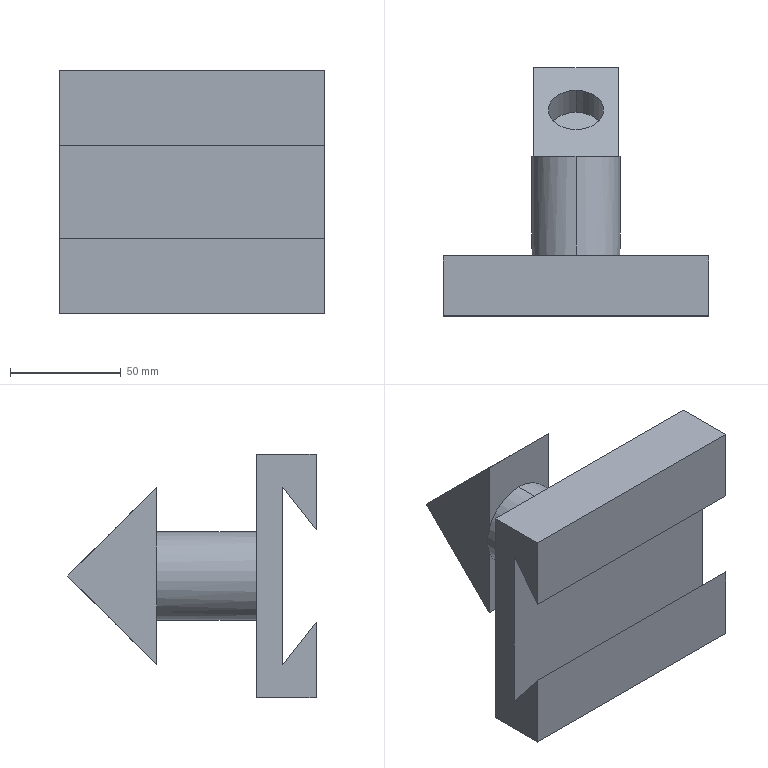Component | SolidWorks | PassiveRollerAssembly-1_DovetailSlot-1 | 1 solid | 26 faces | box 120 x 112 x 110 mm | volume 350204 mm3 | plane 20 | cylinder 6 | commonest cylinder face diameters 25 x4 40 x2
build123d program:
from build123d import *

# Parameters (mm, degrees)
BOSS_EXTRUDE1_DEPTH = 120
SKETCH2_R           = 20
BOSS_EXTRUDE2_DEPTH = 45
BOSS_EXTRUDE3_DEPTH = 19
SKETCH4_R           = 12.5
CUT_EXTRUDE1_DEPTH  = 14


with BuildPart() as part:
    # Sketch1 → Boss-Extrude1 (new body)
    with BuildSketch(Plane.XY):
        Polygon((-55, 0), (55, 0), (55, -27), (21, -27), (40, -12), (-40, -12), (-21, -27), (-55, -27), align=None)
    extrude(amount=BOSS_EXTRUDE1_DEPTH)

    # Sketch2 → Boss-Extrude2 (add)
    with BuildSketch(Plane(origin=(0, 0, 0), x_dir=(1, 0, 0), z_dir=(0, 1, 0))):
        with Locations((0, -60)):
            Circle(SKETCH2_R)
    extrude(amount=BOSS_EXTRUDE2_DEPTH)

    # Sketch3 → Boss-Extrude3 (add, symmetric)
    with BuildSketch(Plane.XY.offset(60)):
        Polygon((-40, 45), (40, 45), (0, 85), align=None)
    extrude(amount=BOSS_EXTRUDE3_DEPTH, both=True)

    # Sketch4 → Cut-Extrude1 (cut)
    with BuildSketch(Plane(origin=(42.5, 42.5, 0), x_dir=(0, 0, -1), z_dir=(0.7071, 0.7071, 0))):
        with Locations(Location((-60, 33.154, 0), (0, 0, 90))):
            Circle(SKETCH4_R)
    cut_extrude1 = extrude(amount=-CUT_EXTRUDE1_DEPTH, mode=Mode.SUBTRACT)

    # Mirror1: Cut-Extrude1 across plane
    add(cut_extrude1.mirror(Plane(origin=(0, 0, 0), x_dir=(0, 0, 1), z_dir=(1, 0, 0))), mode=Mode.SUBTRACT)


solid = part.part

# Placed as in the assembly
solid = solid.moved(Location((2156.026, 589, 269.5), (0, 90, 0)))
STEP:
#1=CARTESIAN_POINT('',(87.245,25.047,11.319));
#2=VERTEX_POINT('',#1);
#3=CARTESIAN_POINT('',(87.245,25.743,10.623));
#4=VERTEX_POINT('',#3);
#5=CARTESIAN_POINT('',(87.245,25.395,10.971));
#6=DIRECTION('',(0.,-0.7071,-0.7071));
#7=DIRECTION('',(0.,0.7071,-0.7071));
#8=AXIS2_PLACEMENT_3D('',#5,#6,#7);
#9=CIRCLE('',#8,0.4921);
#10=EDGE_CURVE('',#2,#4,#9,.T.);
#11=ORIENTED_EDGE('',*,*,#10,.T.);
#12=CARTESIAN_POINT('',(87.245,26.133,11.013));
#13=VERTEX_POINT('',#12);
#14=CARTESIAN_POINT('',(87.245,25.743,10.623));
#15=DIRECTION('',(0.,0.7071,0.7071));
#16=VECTOR('',#15,39.37);
#17=LINE('',#14,#16);
#18=EDGE_CURVE('',#4,#13,#17,.T.);
#19=ORIENTED_EDGE('',*,*,#18,.T.);
#20=CARTESIAN_POINT('',(87.245,25.437,11.708));
#21=VERTEX_POINT('',#20);
#22=CARTESIAN_POINT('',(87.245,25.785,11.36));
#23=DIRECTION('',(0.,-0.7071,-0.7071));
#24=DIRECTION('',(0.,0.7071,-0.7071));
#25=AXIS2_PLACEMENT_3D('',#22,#23,#24);
#26=CIRCLE('',#25,0.4921);
#27=EDGE_CURVE('',#21,#13,#26,.T.);
#28=ORIENTED_EDGE('',*,*,#27,.F.);
#29=CARTESIAN_POINT('',(87.245,25.047,11.319));
#30=DIRECTION('',(0.,0.7071,0.7071));
#31=VECTOR('',#30,39.37);
#32=LINE('',#29,#31);
#33=EDGE_CURVE('',#2,#21,#32,.T.);
#34=ORIENTED_EDGE('',*,*,#33,.F.);
#35=EDGE_LOOP('',(#11,#19,#28,#34));
#36=FACE_OUTER_BOUND('',#35,.T.);
#37=CARTESIAN_POINT('',(87.245,25.395,10.971));
#38=DIRECTION('',(0.,0.7071,0.7071));
#39=DIRECTION('',(0.,-0.7071,0.7071));
#40=AXIS2_PLACEMENT_3D('',#37,#38,#39);
#41=CYLINDRICAL_SURFACE('',#40,0.4921);
#42=ADVANCED_FACE('',(#36),#41,.F.);
#43=CARTESIAN_POINT('',(87.245,25.047,9.902));
#44=VERTEX_POINT('',#43);
#45=CARTESIAN_POINT('',(87.245,25.743,10.598));
#46=VERTEX_POINT('',#45);
#47=CARTESIAN_POINT('',(87.245,25.395,10.25));
#48=DIRECTION('',(0.,0.7071,-0.7071));
#49=DIRECTION('',(0.,0.7071,0.7071));
#50=AXIS2_PLACEMENT_3D('',#47,#48,#49);
#51=CIRCLE('',#50,0.4921);
#52=EDGE_CURVE('',#44,#46,#51,.T.);
#53=ORIENTED_EDGE('',*,*,#52,.F.);
#54=CARTESIAN_POINT('',(87.245,25.437,9.512));
#55=VERTEX_POINT('',#54);
#56=CARTESIAN_POINT('',(87.245,25.047,9.902));
#57=DIRECTION('',(0.,0.7071,-0.7071));
#58=VECTOR('',#57,39.37);
#59=LINE('',#56,#58);
#60=EDGE_CURVE('',#44,#55,#59,.T.);
#61=ORIENTED_EDGE('',*,*,#60,.T.);
#62=CARTESIAN_POINT('',(87.245,26.133,10.208));
#63=VERTEX_POINT('',#62);
#64=CARTESIAN_POINT('',(87.245,25.785,9.86));
#65=DIRECTION('',(0.,0.7071,-0.7071));
#66=DIRECTION('',(0.,0.7071,0.7071));
#67=AXIS2_PLACEMENT_3D('',#64,#65,#66);
#68=CIRCLE('',#67,0.4921);
#69=EDGE_CURVE('',#55,#63,#68,.T.);
#70=ORIENTED_EDGE('',*,*,#69,.T.);
#71=CARTESIAN_POINT('',(87.245,25.743,10.598));
#72=DIRECTION('',(0.,0.7071,-0.7071));
#73=VECTOR('',#72,39.37);
#74=LINE('',#71,#73);
#75=EDGE_CURVE('',#46,#63,#74,.T.);
#76=ORIENTED_EDGE('',*,*,#75,.F.);
#77=EDGE_LOOP('',(#53,#61,#70,#76));
#78=FACE_OUTER_BOUND('',#77,.T.);
#79=CARTESIAN_POINT('',(87.245,25.395,10.25));
#80=DIRECTION('',(0.,0.7071,-0.7071));
#81=DIRECTION('',(0.,0.7071,0.7071));
#82=AXIS2_PLACEMENT_3D('',#79,#80,#81);
#83=CYLINDRICAL_SURFACE('',#82,0.4921);
#84=ADVANCED_FACE('',(#78),#83,.F.);
#85=CARTESIAN_POINT('',(87.245,24.961,11.398));
#86=VERTEX_POINT('',#85);
#87=CARTESIAN_POINT('',(87.993,24.961,10.856));
#88=VERTEX_POINT('',#87);
#89=CARTESIAN_POINT('',(87.245,24.961,10.61));
#90=DIRECTION('',(0.,1.,-0.));
#91=DIRECTION('',(0.,0.,1.));
#92=AXIS2_PLACEMENT_3D('',#89,#90,#91);
#93=CIRCLE('',#92,0.7874);
#94=EDGE_CURVE('',#86,#88,#93,.T.);
#95=ORIENTED_EDGE('',*,*,#94,.F.);
#96=CARTESIAN_POINT('',(87.245,23.189,11.398));
#97=VERTEX_POINT('',#96);
#98=CARTESIAN_POINT('',(87.245,24.961,11.398));
#99=DIRECTION('',(0.,-1.,0.));
#100=VECTOR('',#99,39.37);
#101=LINE('',#98,#100);
#102=EDGE_CURVE('',#86,#97,#101,.T.);
#103=ORIENTED_EDGE('',*,*,#102,.T.);
#104=CARTESIAN_POINT('',(87.245,23.189,9.823));
#105=VERTEX_POINT('',#104);
#106=CARTESIAN_POINT('',(87.245,23.189,10.61));
#107=DIRECTION('',(0.,1.,-0.));
#108=DIRECTION('',(0.,0.,-1.));
#109=AXIS2_PLACEMENT_3D('',#106,#107,#108);
#110=CIRCLE('',#109,0.7874);
#111=EDGE_CURVE('',#97,#105,#110,.T.);
#112=ORIENTED_EDGE('',*,*,#111,.T.);
#113=CARTESIAN_POINT('',(87.245,24.961,9.823));
#114=VERTEX_POINT('',#113);
#115=CARTESIAN_POINT('',(87.245,24.961,9.823));
#116=DIRECTION('',(0.,-1.,0.));
#117=VECTOR('',#116,39.37);
#118=LINE('',#115,#117);
#119=EDGE_CURVE('',#114,#105,#118,.T.);
#120=ORIENTED_EDGE('',*,*,#119,.F.);
#121=CARTESIAN_POINT('',(87.993,24.961,10.364));
#122=VERTEX_POINT('',#121);
#123=CARTESIAN_POINT('',(87.245,24.961,10.61));
#124=DIRECTION('',(0.,1.,-0.));
#125=DIRECTION('',(0.,0.,1.));
#126=AXIS2_PLACEMENT_3D('',#123,#124,#125);
#127=CIRCLE('',#126,0.7874);
#128=EDGE_CURVE('',#122,#114,#127,.T.);
#129=ORIENTED_EDGE('',*,*,#128,.F.);
#130=CARTESIAN_POINT('',(87.245,24.961,10.61));
#131=DIRECTION('',(0.,1.,-0.));
#132=DIRECTION('',(0.,0.,1.));
#133=AXIS2_PLACEMENT_3D('',#130,#131,#132);
#134=CIRCLE('',#133,0.7874);
#135=EDGE_CURVE('',#88,#122,#134,.T.);
#136=ORIENTED_EDGE('',*,*,#135,.F.);
#137=EDGE_LOOP('',(#95,#103,#112,#120,#129,#136));
#138=FACE_OUTER_BOUND('',#137,.T.);
#139=CARTESIAN_POINT('',(87.245,24.961,10.61));
#140=DIRECTION('',(0.,-1.,0.));
#141=DIRECTION('',(0.,0.,-1.));
#142=AXIS2_PLACEMENT_3D('',#139,#140,#141);
#143=CYLINDRICAL_SURFACE('',#142,0.7874);
#144=ADVANCED_FACE('',(#138),#143,.T.);
#145=CARTESIAN_POINT('',(86.497,26.535,10.61));
#146=VERTEX_POINT('',#145);
#147=CARTESIAN_POINT('',(86.497,24.961,12.185));
#148=VERTEX_POINT('',#147);
#149=CARTESIAN_POINT('',(86.497,24.961,12.185));
#150=DIRECTION('',(0.,-0.7071,0.7071));
#151=VECTOR('',#150,39.37);
#152=LINE('',#149,#151);
#153=EDGE_CURVE('',#146,#148,#152,.T.);
#154=ORIENTED_EDGE('',*,*,#153,.T.);
#155=CARTESIAN_POINT('',(87.993,24.961,12.185));
#156=VERTEX_POINT('',#155);
#157=CARTESIAN_POINT('',(87.993,24.961,12.185));
#158=DIRECTION('',(-1.,0.,0.));
#159=VECTOR('',#158,39.37);
#160=LINE('',#157,#159);
#161=EDGE_CURVE('',#156,#148,#160,.T.);
#162=ORIENTED_EDGE('',*,*,#161,.F.);
#163=CARTESIAN_POINT('',(87.993,26.535,10.61));
#164=VERTEX_POINT('',#163);
#165=CARTESIAN_POINT('',(87.993,24.961,12.185));
#166=DIRECTION('',(0.,-0.7071,0.7071));
#167=VECTOR('',#166,39.37);
#168=LINE('',#165,#167);
#169=EDGE_CURVE('',#164,#156,#168,.T.);
#170=ORIENTED_EDGE('',*,*,#169,.F.);
#171=CARTESIAN_POINT('',(87.993,26.535,10.61));
#172=DIRECTION('',(-1.,0.,0.));
#173=VECTOR('',#172,39.37);
#174=LINE('',#171,#173);
#175=EDGE_CURVE('',#164,#146,#174,.T.);
#176=ORIENTED_EDGE('',*,*,#175,.T.);
#177=EDGE_LOOP('',(#154,#162,#170,#176));
#178=FACE_OUTER_BOUND('',#177,.T.);
#179=ORIENTED_EDGE('',*,*,#27,.T.);
#180=CARTESIAN_POINT('',(87.245,25.785,11.36));
#181=DIRECTION('',(0.,-0.7071,-0.7071));
#182=DIRECTION('',(0.,0.7071,-0.7071));
#183=AXIS2_PLACEMENT_3D('',#180,#181,#182);
#184=CIRCLE('',#183,0.4921);
#185=EDGE_CURVE('',#13,#21,#184,.T.);
#186=ORIENTED_EDGE('',*,*,#185,.T.);
#187=EDGE_LOOP('',(#179,#186));
#188=FACE_BOUND('',#187,.T.);
#189=CARTESIAN_POINT('',(87.993,24.961,12.185));
#190=DIRECTION('',(0.,-0.7071,-0.7071));
#191=DIRECTION('',(0.,0.7071,-0.7071));
#192=AXIS2_PLACEMENT_3D('',#189,#190,#191);
#193=PLANE('',#192);
#194=ADVANCED_FACE('',(#178,#188),#193,.F.);
#195=CARTESIAN_POINT('',(86.497,24.961,10.364));
#196=VERTEX_POINT('',#195);
#197=CARTESIAN_POINT('',(86.497,24.961,10.856));
#198=VERTEX_POINT('',#197);
#199=CARTESIAN_POINT('',(87.245,24.961,10.61));
#200=DIRECTION('',(0.,1.,-0.));
#201=DIRECTION('',(0.,0.,1.));
#202=AXIS2_PLACEMENT_3D('',#199,#200,#201);
#203=CIRCLE('',#202,0.7874);
#204=EDGE_CURVE('',#196,#198,#203,.T.);
#205=ORIENTED_EDGE('',*,*,#204,.T.);
#206=CARTESIAN_POINT('',(86.497,24.961,12.185));
#207=DIRECTION('',(0.,-0.,-1.));
#208=VECTOR('',#207,39.37);
#209=LINE('',#206,#208);
#210=EDGE_CURVE('',#198,#196,#209,.T.);
#211=ORIENTED_EDGE('',*,*,#210,.T.);
#212=EDGE_LOOP('',(#205,#211));
#213=FACE_OUTER_BOUND('',#212,.T.);
#214=CARTESIAN_POINT('',(87.245,24.961,10.61));
#215=DIRECTION('',(0.,1.,0.));
#216=DIRECTION('',(0.,-0.,1.));
#217=AXIS2_PLACEMENT_3D('',#214,#215,#216);
#218=PLANE('',#217);
#219=ADVANCED_FACE('',(#213),#218,.T.);
#220=CARTESIAN_POINT('',(84.883,23.189,8.445));
#221=VERTEX_POINT('',#220);
#222=CARTESIAN_POINT('',(84.883,23.189,12.776));
#223=VERTEX_POINT('',#222);
#224=CARTESIAN_POINT('',(84.883,23.189,12.776));
#225=DIRECTION('',(0.,-0.,1.));
#226=VECTOR('',#225,39.37);
#227=LINE('',#224,#226);
#228=EDGE_CURVE('',#221,#223,#227,.T.);
#229=ORIENTED_EDGE('',*,*,#228,.T.);
#230=CARTESIAN_POINT('',(89.607,23.189,12.776));
#231=VERTEX_POINT('',#230);
#232=CARTESIAN_POINT('',(89.607,23.189,12.776));
#233=DIRECTION('',(-1.,0.,0.));
#234=VECTOR('',#233,39.37);
#235=LINE('',#232,#234);
#236=EDGE_CURVE('',#231,#223,#235,.T.);
#237=ORIENTED_EDGE('',*,*,#236,.F.);
#238=CARTESIAN_POINT('',(89.607,23.189,8.445));
#239=VERTEX_POINT('',#238);
#240=CARTESIAN_POINT('',(89.607,23.189,12.776));
#241=DIRECTION('',(0.,-0.,1.));
#242=VECTOR('',#241,39.37);
#243=LINE('',#240,#242);
#244=EDGE_CURVE('',#239,#231,#243,.T.);
#245=ORIENTED_EDGE('',*,*,#244,.F.);
#246=CARTESIAN_POINT('',(89.607,23.189,8.445));
#247=DIRECTION('',(-1.,0.,0.));
#248=VECTOR('',#247,39.37);
#249=LINE('',#246,#248);
#250=EDGE_CURVE('',#239,#221,#249,.T.);
#251=ORIENTED_EDGE('',*,*,#250,.T.);
#252=EDGE_LOOP('',(#229,#237,#245,#251));
#253=FACE_OUTER_BOUND('',#252,.T.);
#254=CARTESIAN_POINT('',(87.245,23.189,10.61));
#255=DIRECTION('',(0.,1.,-0.));
#256=DIRECTION('',(0.,0.,-1.));
#257=AXIS2_PLACEMENT_3D('',#254,#255,#256);
#258=CIRCLE('',#257,0.7874);
#259=EDGE_CURVE('',#105,#97,#258,.T.);
#260=ORIENTED_EDGE('',*,*,#259,.F.);
#261=ORIENTED_EDGE('',*,*,#111,.F.);
#262=EDGE_LOOP('',(#260,#261));
#263=FACE_BOUND('',#262,.T.);
#264=CARTESIAN_POINT('',(89.607,23.189,12.776));
#265=DIRECTION('',(0.,-1.,-0.));
#266=DIRECTION('',(0.,0.,-1.));
#267=AXIS2_PLACEMENT_3D('',#264,#265,#266);
#268=PLANE('',#267);
#269=ADVANCED_FACE('',(#253,#263),#268,.F.);
#270=CARTESIAN_POINT('',(84.883,22.126,8.445));
#271=VERTEX_POINT('',#270);
#272=CARTESIAN_POINT('',(84.883,23.189,8.445));
#273=DIRECTION('',(0.,1.,-0.));
#274=VECTOR('',#273,39.37);
#275=LINE('',#272,#274);
#276=EDGE_CURVE('',#271,#221,#275,.T.);
#277=ORIENTED_EDGE('',*,*,#276,.T.);
#278=ORIENTED_EDGE('',*,*,#250,.F.);
#279=CARTESIAN_POINT('',(89.607,22.126,8.445));
#280=VERTEX_POINT('',#279);
#281=CARTESIAN_POINT('',(89.607,23.189,8.445));
#282=DIRECTION('',(0.,1.,-0.));
#283=VECTOR('',#282,39.37);
#284=LINE('',#281,#283);
#285=EDGE_CURVE('',#280,#239,#284,.T.);
#286=ORIENTED_EDGE('',*,*,#285,.F.);
#287=CARTESIAN_POINT('',(89.607,22.126,8.445));
#288=DIRECTION('',(-1.,0.,0.));
#289=VECTOR('',#288,39.37);
#290=LINE('',#287,#289);
#291=EDGE_CURVE('',#280,#271,#290,.T.);
#292=ORIENTED_EDGE('',*,*,#291,.T.);
#293=EDGE_LOOP('',(#277,#278,#286,#292));
#294=FACE_OUTER_BOUND('',#293,.T.);
#295=CARTESIAN_POINT('',(89.607,23.189,8.445));
#296=DIRECTION('',(0.,0.,1.));
#297=DIRECTION('',(1.,0.,0.));
#298=AXIS2_PLACEMENT_3D('',#295,#296,#297);
#299=PLANE('',#298);
#300=ADVANCED_FACE('',(#294),#299,.F.);
#301=CARTESIAN_POINT('',(84.883,22.126,12.776));
#302=VERTEX_POINT('',#301);
#303=CARTESIAN_POINT('',(84.883,23.189,12.776));
#304=DIRECTION('',(0.,-1.,0.));
#305=VECTOR('',#304,39.37);
#306=LINE('',#303,#305);
#307=EDGE_CURVE('',#223,#302,#306,.T.);
#308=ORIENTED_EDGE('',*,*,#307,.T.);
#309=CARTESIAN_POINT('',(89.607,22.126,12.776));
#310=VERTEX_POINT('',#309);
#311=CARTESIAN_POINT('',(89.607,22.126,12.776));
#312=DIRECTION('',(-1.,0.,0.));
#313=VECTOR('',#312,39.37);
#314=LINE('',#311,#313);
#315=EDGE_CURVE('',#310,#302,#314,.T.);
#316=ORIENTED_EDGE('',*,*,#315,.F.);
#317=CARTESIAN_POINT('',(89.607,23.189,12.776));
#318=DIRECTION('',(0.,-1.,0.));
#319=VECTOR('',#318,39.37);
#320=LINE('',#317,#319);
#321=EDGE_CURVE('',#231,#310,#320,.T.);
#322=ORIENTED_EDGE('',*,*,#321,.F.);
#323=ORIENTED_EDGE('',*,*,#236,.T.);
#324=EDGE_LOOP('',(#308,#316,#322,#323));
#325=FACE_OUTER_BOUND('',#324,.T.);
#326=CARTESIAN_POINT('',(89.607,23.189,12.776));
#327=DIRECTION('',(0.,-0.,-1.));
#328=DIRECTION('',(-1.,0.,0.));
#329=AXIS2_PLACEMENT_3D('',#326,#327,#328);
#330=PLANE('',#329);
#331=ADVANCED_FACE('',(#325),#330,.F.);
#332=CARTESIAN_POINT('',(84.883,22.126,11.437));
#333=VERTEX_POINT('',#332);
#334=CARTESIAN_POINT('',(84.883,22.126,12.776));
#335=DIRECTION('',(0.,-0.,-1.));
#336=VECTOR('',#335,39.37);
#337=LINE('',#334,#336);
#338=EDGE_CURVE('',#302,#333,#337,.T.);
#339=ORIENTED_EDGE('',*,*,#338,.T.);
#340=CARTESIAN_POINT('',(89.607,22.126,11.437));
#341=VERTEX_POINT('',#340);
#342=CARTESIAN_POINT('',(89.607,22.126,11.437));
#343=DIRECTION('',(-1.,0.,0.));
#344=VECTOR('',#343,39.37);
#345=LINE('',#342,#344);
#346=EDGE_CURVE('',#341,#333,#345,.T.);
#347=ORIENTED_EDGE('',*,*,#346,.F.);
#348=CARTESIAN_POINT('',(89.607,22.126,12.776));
#349=DIRECTION('',(0.,-0.,-1.));
#350=VECTOR('',#349,39.37);
#351=LINE('',#348,#350);
#352=EDGE_CURVE('',#310,#341,#351,.T.);
#353=ORIENTED_EDGE('',*,*,#352,.F.);
#354=ORIENTED_EDGE('',*,*,#315,.T.);
#355=EDGE_LOOP('',(#339,#347,#353,#354));
#356=FACE_OUTER_BOUND('',#355,.T.);
#357=CARTESIAN_POINT('',(89.607,22.126,12.776));
#358=DIRECTION('',(0.,1.,-0.));
#359=DIRECTION('',(0.,0.,1.));
#360=AXIS2_PLACEMENT_3D('',#357,#358,#359);
#361=PLANE('',#360);
#362=ADVANCED_FACE('',(#356),#361,.F.);
#363=CARTESIAN_POINT('',(84.883,22.717,12.185));
#364=VERTEX_POINT('',#363);
#365=CARTESIAN_POINT('',(84.883,22.126,11.437));
#366=DIRECTION('',(0.,0.6196,0.7849));
#367=VECTOR('',#366,39.37);
#368=LINE('',#365,#367);
#369=EDGE_CURVE('',#333,#364,#368,.T.);
#370=ORIENTED_EDGE('',*,*,#369,.T.);
#371=CARTESIAN_POINT('',(89.607,22.717,12.185));
#372=VERTEX_POINT('',#371);
#373=CARTESIAN_POINT('',(89.607,22.717,12.185));
#374=DIRECTION('',(-1.,0.,0.));
#375=VECTOR('',#374,39.37);
#376=LINE('',#373,#375);
#377=EDGE_CURVE('',#372,#364,#376,.T.);
#378=ORIENTED_EDGE('',*,*,#377,.F.);
#379=CARTESIAN_POINT('',(89.607,22.126,11.437));
#380=DIRECTION('',(0.,0.6196,0.7849));
#381=VECTOR('',#380,39.37);
#382=LINE('',#379,#381);
#383=EDGE_CURVE('',#341,#372,#382,.T.);
#384=ORIENTED_EDGE('',*,*,#383,.F.);
#385=ORIENTED_EDGE('',*,*,#346,.T.);
#386=EDGE_LOOP('',(#370,#378,#384,#385));
#387=FACE_OUTER_BOUND('',#386,.T.);
#388=CARTESIAN_POINT('',(89.607,22.126,11.437));
#389=DIRECTION('',(0.,-0.7849,0.6196));
#390=DIRECTION('',(0.,-0.6196,-0.7849));
#391=AXIS2_PLACEMENT_3D('',#388,#389,#390);
#392=PLANE('',#391);
#393=ADVANCED_FACE('',(#387),#392,.F.);
#394=CARTESIAN_POINT('',(84.883,22.717,9.035));
#395=VERTEX_POINT('',#394);
#396=CARTESIAN_POINT('',(84.883,22.717,9.035));
#397=DIRECTION('',(0.,0.,-1.));
#398=VECTOR('',#397,39.37);
#399=LINE('',#396,#398);
#400=EDGE_CURVE('',#364,#395,#399,.T.);
#401=ORIENTED_EDGE('',*,*,#400,.T.);
#402=CARTESIAN_POINT('',(89.607,22.717,9.035));
#403=VERTEX_POINT('',#402);
#404=CARTESIAN_POINT('',(89.607,22.717,9.035));
#405=DIRECTION('',(-1.,0.,0.));
#406=VECTOR('',#405,39.37);
#407=LINE('',#404,#406);
#408=EDGE_CURVE('',#403,#395,#407,.T.);
#409=ORIENTED_EDGE('',*,*,#408,.F.);
#410=CARTESIAN_POINT('',(89.607,22.717,9.035));
#411=DIRECTION('',(0.,0.,-1.));
#412=VECTOR('',#411,39.37);
#413=LINE('',#410,#412);
#414=EDGE_CURVE('',#372,#403,#413,.T.);
#415=ORIENTED_EDGE('',*,*,#414,.F.);
#416=ORIENTED_EDGE('',*,*,#377,.T.);
#417=EDGE_LOOP('',(#401,#409,#415,#416));
#418=FACE_OUTER_BOUND('',#417,.T.);
#419=CARTESIAN_POINT('',(89.607,22.717,9.035));
#420=DIRECTION('',(0.,1.,0.));
#421=DIRECTION('',(0.,-0.,1.));
#422=AXIS2_PLACEMENT_3D('',#419,#420,#421);
#423=PLANE('',#422);
#424=ADVANCED_FACE('',(#418),#423,.F.);
#425=CARTESIAN_POINT('',(84.883,22.126,9.783));
#426=VERTEX_POINT('',#425);
#427=CARTESIAN_POINT('',(84.883,22.126,9.783));
#428=DIRECTION('',(0.,-0.6196,0.7849));
#429=VECTOR('',#428,39.37);
#430=LINE('',#427,#429);
#431=EDGE_CURVE('',#395,#426,#430,.T.);
#432=ORIENTED_EDGE('',*,*,#431,.T.);
#433=CARTESIAN_POINT('',(89.607,22.126,9.783));
#434=VERTEX_POINT('',#433);
#435=CARTESIAN_POINT('',(89.607,22.126,9.783));
#436=DIRECTION('',(-1.,0.,0.));
#437=VECTOR('',#436,39.37);
#438=LINE('',#435,#437);
#439=EDGE_CURVE('',#434,#426,#438,.T.);
#440=ORIENTED_EDGE('',*,*,#439,.F.);
#441=CARTESIAN_POINT('',(89.607,22.126,9.783));
#442=DIRECTION('',(0.,-0.6196,0.7849));
#443=VECTOR('',#442,39.37);
#444=LINE('',#441,#443);
#445=EDGE_CURVE('',#403,#434,#444,.T.);
#446=ORIENTED_EDGE('',*,*,#445,.F.);
#447=ORIENTED_EDGE('',*,*,#408,.T.);
#448=EDGE_LOOP('',(#432,#440,#446,#447));
#449=FACE_OUTER_BOUND('',#448,.T.);
#450=CARTESIAN_POINT('',(89.607,22.126,9.783));
#451=DIRECTION('',(0.,-0.7849,-0.6196));
#452=DIRECTION('',(0.,0.6196,-0.7849));
#453=AXIS2_PLACEMENT_3D('',#450,#451,#452);
#454=PLANE('',#453);
#455=ADVANCED_FACE('',(#449),#454,.F.);
#456=CARTESIAN_POINT('',(84.883,22.126,8.445));
#457=DIRECTION('',(0.,0.,-1.));
#458=VECTOR('',#457,39.37);
#459=LINE('',#456,#458);
#460=EDGE_CURVE('',#426,#271,#459,.T.);
#461=ORIENTED_EDGE('',*,*,#460,.T.);
#462=ORIENTED_EDGE('',*,*,#291,.F.);
#463=CARTESIAN_POINT('',(89.607,22.126,8.445));
#464=DIRECTION('',(0.,0.,-1.));
#465=VECTOR('',#464,39.37);
#466=LINE('',#463,#465);
#467=EDGE_CURVE('',#434,#280,#466,.T.);
#468=ORIENTED_EDGE('',*,*,#467,.F.);
#469=ORIENTED_EDGE('',*,*,#439,.T.);
#470=EDGE_LOOP('',(#461,#462,#468,#469));
#471=FACE_OUTER_BOUND('',#470,.T.);
#472=CARTESIAN_POINT('',(89.607,22.126,8.445));
#473=DIRECTION('',(0.,1.,0.));
#474=DIRECTION('',(0.,-0.,1.));
#475=AXIS2_PLACEMENT_3D('',#472,#473,#474);
#476=PLANE('',#475);
#477=ADVANCED_FACE('',(#471),#476,.F.);
#478=ORIENTED_EDGE('',*,*,#285,.T.);
#479=ORIENTED_EDGE('',*,*,#244,.T.);
#480=ORIENTED_EDGE('',*,*,#321,.T.);
#481=ORIENTED_EDGE('',*,*,#352,.T.);
#482=ORIENTED_EDGE('',*,*,#383,.T.);
#483=ORIENTED_EDGE('',*,*,#414,.T.);
#484=ORIENTED_EDGE('',*,*,#445,.T.);
#485=ORIENTED_EDGE('',*,*,#467,.T.);
#486=EDGE_LOOP('',(#478,#479,#480,#481,#482,#483,#484,#485));
#487=FACE_OUTER_BOUND('',#486,.T.);
#488=CARTESIAN_POINT('',(89.607,23.189,10.61));
#489=DIRECTION('',(-1.,0.,0.));
#490=DIRECTION('',(0.,0.,1.));
#491=AXIS2_PLACEMENT_3D('',#488,#489,#490);
#492=PLANE('',#491);
#493=ADVANCED_FACE('',(#487),#492,.F.);
#494=ORIENTED_EDGE('',*,*,#276,.F.);
#495=ORIENTED_EDGE('',*,*,#460,.F.);
#496=ORIENTED_EDGE('',*,*,#431,.F.);
#497=ORIENTED_EDGE('',*,*,#400,.F.);
#498=ORIENTED_EDGE('',*,*,#369,.F.);
#499=ORIENTED_EDGE('',*,*,#338,.F.);
#500=ORIENTED_EDGE('',*,*,#307,.F.);
#501=ORIENTED_EDGE('',*,*,#228,.F.);
#502=EDGE_LOOP('',(#494,#495,#496,#497,#498,#499,#500,#501));
#503=FACE_OUTER_BOUND('',#502,.T.);
#504=CARTESIAN_POINT('',(84.883,23.189,10.61));
#505=DIRECTION('',(-1.,0.,0.));
#506=DIRECTION('',(0.,0.,1.));
#507=AXIS2_PLACEMENT_3D('',#504,#505,#506);
#508=PLANE('',#507);
#509=ADVANCED_FACE('',(#503),#508,.T.);
#510=ORIENTED_EDGE('',*,*,#102,.F.);
#511=CARTESIAN_POINT('',(87.245,24.961,10.61));
#512=DIRECTION('',(0.,1.,-0.));
#513=DIRECTION('',(0.,0.,1.));
#514=AXIS2_PLACEMENT_3D('',#511,#512,#513);
#515=CIRCLE('',#514,0.7874);
#516=EDGE_CURVE('',#198,#86,#515,.T.);
#517=ORIENTED_EDGE('',*,*,#516,.F.);
#518=ORIENTED_EDGE('',*,*,#204,.F.);
#519=CARTESIAN_POINT('',(87.245,24.961,10.61));
#520=DIRECTION('',(0.,1.,-0.));
#521=DIRECTION('',(0.,0.,1.));
#522=AXIS2_PLACEMENT_3D('',#519,#520,#521);
#523=CIRCLE('',#522,0.7874);
#524=EDGE_CURVE('',#114,#196,#523,.T.);
#525=ORIENTED_EDGE('',*,*,#524,.F.);
#526=ORIENTED_EDGE('',*,*,#119,.T.);
#527=ORIENTED_EDGE('',*,*,#259,.T.);
#528=EDGE_LOOP('',(#510,#517,#518,#525,#526,#527));
#529=FACE_OUTER_BOUND('',#528,.T.);
#530=CARTESIAN_POINT('',(87.245,24.961,10.61));
#531=DIRECTION('',(0.,-1.,0.));
#532=DIRECTION('',(0.,0.,-1.));
#533=AXIS2_PLACEMENT_3D('',#530,#531,#532);
#534=CYLINDRICAL_SURFACE('',#533,0.7874);
#535=ADVANCED_FACE('',(#529),#534,.T.);
#536=CARTESIAN_POINT('',(87.993,24.961,12.185));
#537=DIRECTION('',(0.,-0.,-1.));
#538=VECTOR('',#537,39.37);
#539=LINE('',#536,#538);
#540=EDGE_CURVE('',#88,#122,#539,.T.);
#541=ORIENTED_EDGE('',*,*,#540,.F.);
#542=ORIENTED_EDGE('',*,*,#135,.T.);
#543=EDGE_LOOP('',(#541,#542));
#544=FACE_OUTER_BOUND('',#543,.T.);
#545=CARTESIAN_POINT('',(87.245,24.961,10.61));
#546=DIRECTION('',(0.,1.,0.));
#547=DIRECTION('',(0.,-0.,1.));
#548=AXIS2_PLACEMENT_3D('',#545,#546,#547);
#549=PLANE('',#548);
#550=ADVANCED_FACE('',(#544),#549,.T.);
#551=CARTESIAN_POINT('',(87.993,24.961,9.035));
#552=VERTEX_POINT('',#551);
#553=CARTESIAN_POINT('',(87.993,24.961,12.185));
#554=DIRECTION('',(0.,-0.,-1.));
#555=VECTOR('',#554,39.37);
#556=LINE('',#553,#555);
#557=EDGE_CURVE('',#122,#552,#556,.T.);
#558=ORIENTED_EDGE('',*,*,#557,.F.);
#559=ORIENTED_EDGE('',*,*,#128,.T.);
#560=ORIENTED_EDGE('',*,*,#524,.T.);
#561=CARTESIAN_POINT('',(86.497,24.961,9.035));
#562=VERTEX_POINT('',#561);
#563=CARTESIAN_POINT('',(86.497,24.961,12.185));
#564=DIRECTION('',(0.,-0.,-1.));
#565=VECTOR('',#564,39.37);
#566=LINE('',#563,#565);
#567=EDGE_CURVE('',#196,#562,#566,.T.);
#568=ORIENTED_EDGE('',*,*,#567,.T.);
#569=CARTESIAN_POINT('',(87.993,24.961,9.035));
#570=DIRECTION('',(-1.,0.,0.));
#571=VECTOR('',#570,39.37);
#572=LINE('',#569,#571);
#573=EDGE_CURVE('',#552,#562,#572,.T.);
#574=ORIENTED_EDGE('',*,*,#573,.F.);
#575=EDGE_LOOP('',(#558,#559,#560,#568,#574));
#576=FACE_OUTER_BOUND('',#575,.T.);
#577=CARTESIAN_POINT('',(87.993,24.961,12.185));
#578=DIRECTION('',(0.,1.,-0.));
#579=DIRECTION('',(1.,0.,0.));
#580=AXIS2_PLACEMENT_3D('',#577,#578,#579);
#581=PLANE('',#580);
#582=ADVANCED_FACE('',(#576),#581,.F.);
#583=CARTESIAN_POINT('',(86.497,24.961,12.185));
#584=DIRECTION('',(0.,-0.,-1.));
#585=VECTOR('',#584,39.37);
#586=LINE('',#583,#585);
#587=EDGE_CURVE('',#148,#198,#586,.T.);
#588=ORIENTED_EDGE('',*,*,#587,.T.);
#589=ORIENTED_EDGE('',*,*,#516,.T.);
#590=ORIENTED_EDGE('',*,*,#94,.T.);
#591=CARTESIAN_POINT('',(87.993,24.961,12.185));
#592=DIRECTION('',(0.,-0.,-1.));
#593=VECTOR('',#592,39.37);
#594=LINE('',#591,#593);
#595=EDGE_CURVE('',#156,#88,#594,.T.);
#596=ORIENTED_EDGE('',*,*,#595,.F.);
#597=ORIENTED_EDGE('',*,*,#161,.T.);
#598=EDGE_LOOP('',(#588,#589,#590,#596,#597));
#599=FACE_OUTER_BOUND('',#598,.T.);
#600=CARTESIAN_POINT('',(87.993,24.961,12.185));
#601=DIRECTION('',(0.,1.,-0.));
#602=DIRECTION('',(1.,0.,0.));
#603=AXIS2_PLACEMENT_3D('',#600,#601,#602);
#604=PLANE('',#603);
#605=ADVANCED_FACE('',(#599),#604,.F.);
#606=CARTESIAN_POINT('',(87.245,25.785,9.86));
#607=DIRECTION('',(0.,0.7071,-0.7071));
#608=DIRECTION('',(0.,0.7071,0.7071));
#609=AXIS2_PLACEMENT_3D('',#606,#607,#608);
#610=CIRCLE('',#609,0.4921);
#611=EDGE_CURVE('',#63,#55,#610,.T.);
#612=ORIENTED_EDGE('',*,*,#611,.F.);
#613=ORIENTED_EDGE('',*,*,#69,.F.);
#614=EDGE_LOOP('',(#612,#613));
#615=FACE_BOUND('',#614,.T.);
#616=CARTESIAN_POINT('',(86.497,24.961,9.035));
#617=DIRECTION('',(0.,0.7071,0.7071));
#618=VECTOR('',#617,39.37);
#619=LINE('',#616,#618);
#620=EDGE_CURVE('',#562,#146,#619,.T.);
#621=ORIENTED_EDGE('',*,*,#620,.T.);
#622=ORIENTED_EDGE('',*,*,#175,.F.);
#623=CARTESIAN_POINT('',(87.993,24.961,9.035));
#624=DIRECTION('',(0.,0.7071,0.7071));
#625=VECTOR('',#624,39.37);
#626=LINE('',#623,#625);
#627=EDGE_CURVE('',#552,#164,#626,.T.);
#628=ORIENTED_EDGE('',*,*,#627,.F.);
#629=ORIENTED_EDGE('',*,*,#573,.T.);
#630=EDGE_LOOP('',(#621,#622,#628,#629));
#631=FACE_OUTER_BOUND('',#630,.T.);
#632=CARTESIAN_POINT('',(87.993,24.961,9.035));
#633=DIRECTION('',(0.,-0.7071,0.7071));
#634=DIRECTION('',(0.,-0.7071,-0.7071));
#635=AXIS2_PLACEMENT_3D('',#632,#633,#634);
#636=PLANE('',#635);
#637=ADVANCED_FACE('',(#615,#631),#636,.F.);
#638=ORIENTED_EDGE('',*,*,#627,.T.);
#639=ORIENTED_EDGE('',*,*,#169,.T.);
#640=ORIENTED_EDGE('',*,*,#595,.T.);
#641=ORIENTED_EDGE('',*,*,#540,.T.);
#642=ORIENTED_EDGE('',*,*,#557,.T.);
#643=EDGE_LOOP('',(#638,#639,#640,#641,#642));
#644=FACE_OUTER_BOUND('',#643,.T.);
#645=CARTESIAN_POINT('',(87.993,23.189,10.61));
#646=DIRECTION('',(-1.,0.,0.));
#647=DIRECTION('',(0.,0.,1.));
#648=AXIS2_PLACEMENT_3D('',#645,#646,#647);
#649=PLANE('',#648);
#650=ADVANCED_FACE('',(#644),#649,.F.);
#651=ORIENTED_EDGE('',*,*,#620,.F.);
#652=ORIENTED_EDGE('',*,*,#567,.F.);
#653=ORIENTED_EDGE('',*,*,#210,.F.);
#654=ORIENTED_EDGE('',*,*,#587,.F.);
#655=ORIENTED_EDGE('',*,*,#153,.F.);
#656=EDGE_LOOP('',(#651,#652,#653,#654,#655));
#657=FACE_OUTER_BOUND('',#656,.T.);
#658=CARTESIAN_POINT('',(86.497,23.189,10.61));
#659=DIRECTION('',(-1.,0.,0.));
#660=DIRECTION('',(0.,0.,1.));
#661=AXIS2_PLACEMENT_3D('',#658,#659,#660);
#662=PLANE('',#661);
#663=ADVANCED_FACE('',(#657),#662,.T.);
#664=ORIENTED_EDGE('',*,*,#60,.F.);
#665=CARTESIAN_POINT('',(87.245,25.395,10.25));
#666=DIRECTION('',(0.,0.7071,-0.7071));
#667=DIRECTION('',(0.,0.7071,0.7071));
#668=AXIS2_PLACEMENT_3D('',#665,#666,#667);
#669=CIRCLE('',#668,0.4921);
#670=EDGE_CURVE('',#46,#44,#669,.T.);
#671=ORIENTED_EDGE('',*,*,#670,.F.);
#672=ORIENTED_EDGE('',*,*,#75,.T.);
#673=ORIENTED_EDGE('',*,*,#611,.T.);
#674=EDGE_LOOP('',(#664,#671,#672,#673));
#675=FACE_OUTER_BOUND('',#674,.T.);
#676=CARTESIAN_POINT('',(87.245,25.395,10.25));
#677=DIRECTION('',(0.,0.7071,-0.7071));
#678=DIRECTION('',(0.,0.7071,0.7071));
#679=AXIS2_PLACEMENT_3D('',#676,#677,#678);
#680=CYLINDRICAL_SURFACE('',#679,0.4921);
#681=ADVANCED_FACE('',(#675),#680,.F.);
#682=ORIENTED_EDGE('',*,*,#670,.T.);
#683=ORIENTED_EDGE('',*,*,#52,.T.);
#684=EDGE_LOOP('',(#682,#683));
#685=FACE_OUTER_BOUND('',#684,.T.);
#686=CARTESIAN_POINT('',(87.245,25.395,10.25));
#687=DIRECTION('',(0.,0.7071,-0.7071));
#688=DIRECTION('',(0.,0.7071,0.7071));
#689=AXIS2_PLACEMENT_3D('',#686,#687,#688);
#690=PLANE('',#689);
#691=ADVANCED_FACE('',(#685),#690,.T.);
#692=ORIENTED_EDGE('',*,*,#18,.F.);
#693=CARTESIAN_POINT('',(87.245,25.395,10.971));
#694=DIRECTION('',(0.,-0.7071,-0.7071));
#695=DIRECTION('',(0.,0.7071,-0.7071));
#696=AXIS2_PLACEMENT_3D('',#693,#694,#695);
#697=CIRCLE('',#696,0.4921);
#698=EDGE_CURVE('',#4,#2,#697,.T.);
#699=ORIENTED_EDGE('',*,*,#698,.T.);
#700=ORIENTED_EDGE('',*,*,#33,.T.);
#701=ORIENTED_EDGE('',*,*,#185,.F.);
#702=EDGE_LOOP('',(#692,#699,#700,#701));
#703=FACE_OUTER_BOUND('',#702,.T.);
#704=CARTESIAN_POINT('',(87.245,25.395,10.971));
#705=DIRECTION('',(0.,0.7071,0.7071));
#706=DIRECTION('',(0.,-0.7071,0.7071));
#707=AXIS2_PLACEMENT_3D('',#704,#705,#706);
#708=CYLINDRICAL_SURFACE('',#707,0.4921);
#709=ADVANCED_FACE('',(#703),#708,.F.);
#710=ORIENTED_EDGE('',*,*,#10,.F.);
#711=ORIENTED_EDGE('',*,*,#698,.F.);
#712=EDGE_LOOP('',(#710,#711));
#713=FACE_OUTER_BOUND('',#712,.T.);
#714=CARTESIAN_POINT('',(87.245,25.395,10.971));
#715=DIRECTION('',(0.,0.7071,0.7071));
#716=DIRECTION('',(0.,0.7071,-0.7071));
#717=AXIS2_PLACEMENT_3D('',#714,#715,#716);
#718=PLANE('',#717);
#719=ADVANCED_FACE('',(#713),#718,.T.);
#720=CLOSED_SHELL('',(#42,#84,#144,#194,#219,#269,#300,#331,#362,#393,#424,#455,#477,#493,#509,#535,#550,#582,#605,#637,#650,#663,#681,#691,#709,#719));
#721=MANIFOLD_SOLID_BREP('',#720);
#722=CARTESIAN_POINT('',(0.,0.,0.));
#723=DIRECTION('',(0.,0.,1.));
#724=DIRECTION('',(1.,0.,0.));
#725=AXIS2_PLACEMENT_3D('',#722,#723,#724);
#726=(LENGTH_UNIT()NAMED_UNIT(*)SI_UNIT($,.METRE.));
#727=LENGTH_MEASURE_WITH_UNIT(LENGTH_MEASURE(0.0254),#726);
#728=DIMENSIONAL_EXPONENTS(1.,0.,0.,0.,0.,0.,0.);
#729=(CONVERSION_BASED_UNIT('',#727)LENGTH_UNIT()NAMED_UNIT(#728));
#730=UNCERTAINTY_MEASURE_WITH_UNIT(LENGTH_MEASURE(0.00001),#729,'','');
#731=(NAMED_UNIT(*)PLANE_ANGLE_UNIT()SI_UNIT($,.RADIAN.));
#732=(NAMED_UNIT(*)SI_UNIT($,.STERADIAN.)SOLID_ANGLE_UNIT());
#733=(GEOMETRIC_REPRESENTATION_CONTEXT(3)GLOBAL_UNCERTAINTY_ASSIGNED_CONTEXT((#730))GLOBAL_UNIT_ASSIGNED_CONTEXT((#729,#731,#732))REPRESENTATION_CONTEXT('',''));
#734=ADVANCED_BREP_SHAPE_REPRESENTATION('',(#721,#725),#733);
#735=COLOUR_RGB('',0.7922,0.8196,0.9333);
#736=FILL_AREA_STYLE_COLOUR('',#735);
#737=FILL_AREA_STYLE('',(#736));
#738=SURFACE_STYLE_FILL_AREA(#737);
#739=SURFACE_SIDE_STYLE('',(#738));
#740=SURFACE_STYLE_USAGE(.BOTH.,#739);
#741=PRESENTATION_STYLE_ASSIGNMENT((#740));
#742=STYLED_ITEM('',(#741),#721);
#743=PRESENTATION_LAYER_ASSIGNMENT('','',(#742));
#744=(LENGTH_UNIT()NAMED_UNIT(*)SI_UNIT($,.METRE.));
#745=LENGTH_MEASURE_WITH_UNIT(LENGTH_MEASURE(0.0254),#744);
#746=DIMENSIONAL_EXPONENTS(1.,0.,0.,0.,0.,0.,0.);
#747=(CONVERSION_BASED_UNIT('',#745)LENGTH_UNIT()NAMED_UNIT(#746));
#748=UNCERTAINTY_MEASURE_WITH_UNIT(LENGTH_MEASURE(0.00001),#747,'','');
#749=(NAMED_UNIT(*)PLANE_ANGLE_UNIT()SI_UNIT($,.RADIAN.));
#750=(NAMED_UNIT(*)SI_UNIT($,.STERADIAN.)SOLID_ANGLE_UNIT());
#751=(GEOMETRIC_REPRESENTATION_CONTEXT(3)GLOBAL_UNCERTAINTY_ASSIGNED_CONTEXT((#748))GLOBAL_UNIT_ASSIGNED_CONTEXT((#747,#749,#750))REPRESENTATION_CONTEXT('',''));
#752=MECHANICAL_DESIGN_GEOMETRIC_PRESENTATION_REPRESENTATION('',(#742),#751);